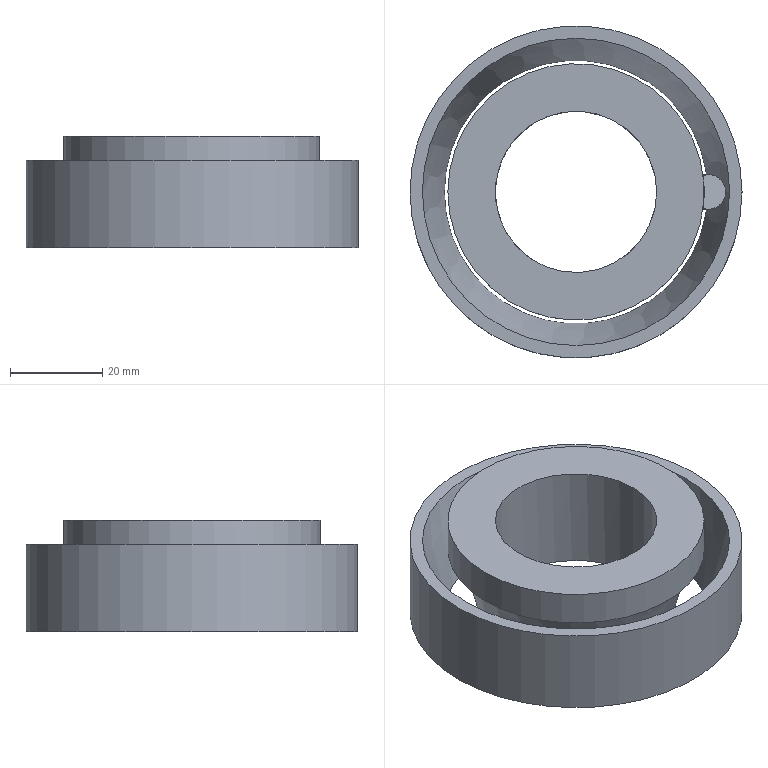Component | NX | CT-ZHOU5-ZHOUCHENG1 | 3 solids | 16 faces | volume 42759 mm3 | plane 6 | cylinder 6 | cone 4 | commonest cylinder face diameters 55.587 x3 7.457 x1 35 x1 72 x1